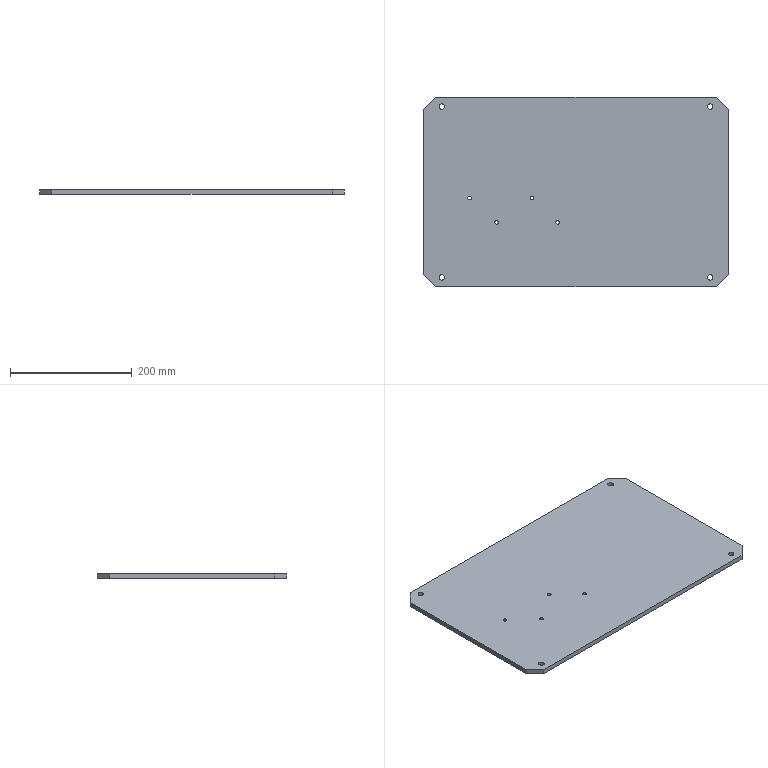Component | SolidWorks | FixedPlateB-1 | 1 solid | 34 faces | volume 1230659 mm3 | cylinder 16 | plane 10 | cone 8 | commonest cylinder face diameters 6 x8 9 x8